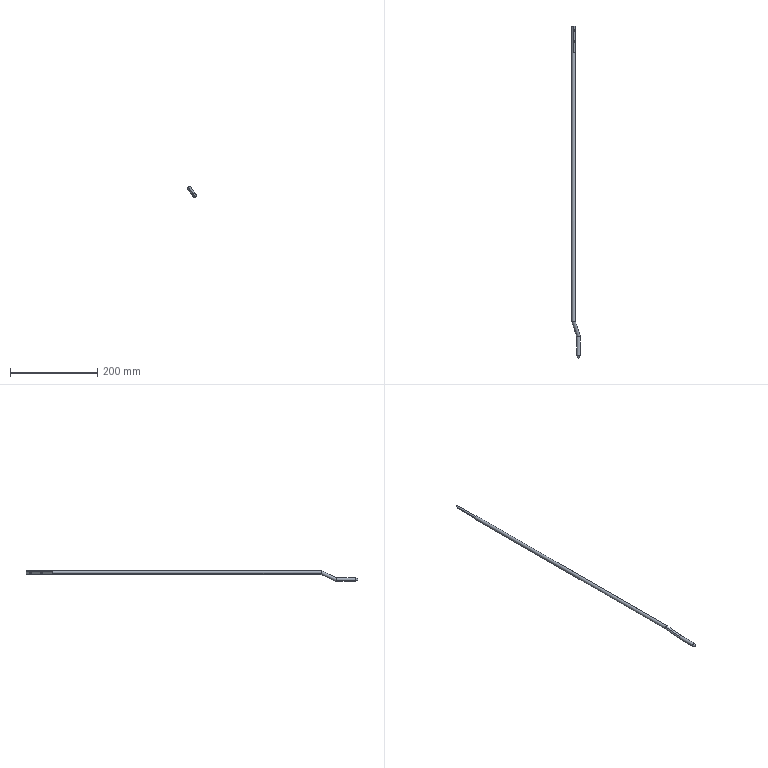Component | SolidWorks | LowerLockRod-1 | 1 solid | 18 faces | box 19.33 x 759.12 x 24.12 mm | volume 36946 mm3 | cylinder 10 | plane 6 | cone 2 | commonest cylinder face diameters 8 x6 4.2 x4
STEP:
#1=CARTESIAN_POINT('',(-12.508,-9.166,84.754));
#2=VERTEX_POINT('',#1);
#3=CARTESIAN_POINT('',(-12.508,-9.332,84.754));
#4=VERTEX_POINT('',#3);
#5=CARTESIAN_POINT('',(-12.508,-9.249,84.754));
#6=DIRECTION('',(-0.818,-0.,-0.5751));
#7=DIRECTION('',(0.,-1.,0.));
#8=AXIS2_PLACEMENT_3D('',#5,#6,#7);
#9=CIRCLE('',#8,0.08268);
#10=EDGE_CURVE('',#2,#4,#9,.T.);
#11=ORIENTED_EDGE('',*,*,#10,.F.);
#12=CARTESIAN_POINT('',(-12.637,-9.166,84.663));
#13=VERTEX_POINT('',#12);
#14=CARTESIAN_POINT('',(-10.705,-9.166,86.022));
#15=DIRECTION('',(-0.818,-0.,-0.5751));
#16=VECTOR('',#15,39.37);
#17=LINE('',#14,#16);
#18=EDGE_CURVE('',#2,#13,#17,.T.);
#19=ORIENTED_EDGE('',*,*,#18,.T.);
#20=CARTESIAN_POINT('',(-12.637,-9.332,84.663));
#21=VERTEX_POINT('',#20);
#22=CARTESIAN_POINT('',(-12.637,-9.249,84.663));
#23=DIRECTION('',(-0.818,-0.,-0.5751));
#24=DIRECTION('',(0.,-1.,0.));
#25=AXIS2_PLACEMENT_3D('',#22,#23,#24);
#26=CIRCLE('',#25,0.08268);
#27=EDGE_CURVE('',#13,#21,#26,.T.);
#28=ORIENTED_EDGE('',*,*,#27,.T.);
#29=CARTESIAN_POINT('',(-10.705,-9.332,86.022));
#30=DIRECTION('',(-0.818,-0.,-0.5751));
#31=VECTOR('',#30,39.37);
#32=LINE('',#29,#31);
#33=EDGE_CURVE('',#4,#21,#32,.T.);
#34=ORIENTED_EDGE('',*,*,#33,.F.);
#35=EDGE_LOOP('',(#11,#19,#28,#34));
#36=FACE_OUTER_BOUND('',#35,.T.);
#37=CARTESIAN_POINT('',(-10.705,-9.249,86.022));
#38=DIRECTION('',(-0.818,-0.,-0.5751));
#39=DIRECTION('',(0.,-1.,0.));
#40=AXIS2_PLACEMENT_3D('',#37,#38,#39);
#41=CYLINDRICAL_SURFACE('',#40,0.08268);
#42=ADVANCED_FACE('',(#36),#41,.F.);
#43=CARTESIAN_POINT('',(-12.508,-8.182,84.754));
#44=VERTEX_POINT('',#43);
#45=CARTESIAN_POINT('',(-12.508,-8.348,84.754));
#46=VERTEX_POINT('',#45);
#47=CARTESIAN_POINT('',(-12.508,-8.265,84.754));
#48=DIRECTION('',(-0.818,-0.,-0.5751));
#49=DIRECTION('',(0.,-1.,0.));
#50=AXIS2_PLACEMENT_3D('',#47,#48,#49);
#51=CIRCLE('',#50,0.08268);
#52=EDGE_CURVE('',#44,#46,#51,.T.);
#53=ORIENTED_EDGE('',*,*,#52,.F.);
#54=CARTESIAN_POINT('',(-12.637,-8.182,84.663));
#55=VERTEX_POINT('',#54);
#56=CARTESIAN_POINT('',(-10.705,-8.182,86.022));
#57=DIRECTION('',(-0.818,-0.,-0.5751));
#58=VECTOR('',#57,39.37);
#59=LINE('',#56,#58);
#60=EDGE_CURVE('',#44,#55,#59,.T.);
#61=ORIENTED_EDGE('',*,*,#60,.T.);
#62=CARTESIAN_POINT('',(-12.637,-8.348,84.663));
#63=VERTEX_POINT('',#62);
#64=CARTESIAN_POINT('',(-12.637,-8.265,84.663));
#65=DIRECTION('',(-0.818,-0.,-0.5751));
#66=DIRECTION('',(0.,-1.,0.));
#67=AXIS2_PLACEMENT_3D('',#64,#65,#66);
#68=CIRCLE('',#67,0.08268);
#69=EDGE_CURVE('',#55,#63,#68,.T.);
#70=ORIENTED_EDGE('',*,*,#69,.T.);
#71=CARTESIAN_POINT('',(-10.705,-8.348,86.022));
#72=DIRECTION('',(-0.818,-0.,-0.5751));
#73=VECTOR('',#72,39.37);
#74=LINE('',#71,#73);
#75=EDGE_CURVE('',#46,#63,#74,.T.);
#76=ORIENTED_EDGE('',*,*,#75,.F.);
#77=EDGE_LOOP('',(#53,#61,#70,#76));
#78=FACE_OUTER_BOUND('',#77,.T.);
#79=CARTESIAN_POINT('',(-10.705,-8.265,86.022));
#80=DIRECTION('',(-0.818,-0.,-0.5751));
#81=DIRECTION('',(0.,-1.,0.));
#82=AXIS2_PLACEMENT_3D('',#79,#80,#81);
#83=CYLINDRICAL_SURFACE('',#82,0.08268);
#84=ADVANCED_FACE('',(#78),#83,.F.);
#85=CARTESIAN_POINT('',(-12.11,-37.758,84.085));
#86=VERTEX_POINT('',#85);
#87=CARTESIAN_POINT('',(-12.143,-37.758,84.063));
#88=VERTEX_POINT('',#87);
#89=CARTESIAN_POINT('',(-12.127,-37.758,84.074));
#90=DIRECTION('',(0.,-1.,-0.));
#91=DIRECTION('',(0.818,0.,0.5751));
#92=AXIS2_PLACEMENT_3D('',#89,#90,#91);
#93=CIRCLE('',#92,0.01969);
#94=EDGE_CURVE('',#86,#88,#93,.T.);
#95=ORIENTED_EDGE('',*,*,#94,.F.);
#96=CARTESIAN_POINT('',(-11.998,-37.522,84.164));
#97=VERTEX_POINT('',#96);
#98=CARTESIAN_POINT('',(-12.11,-37.758,84.085));
#99=DIRECTION('',(0.4122,0.8638,0.2898));
#100=VECTOR('',#99,39.37);
#101=LINE('',#98,#100);
#102=EDGE_CURVE('',#86,#97,#101,.T.);
#103=ORIENTED_EDGE('',*,*,#102,.T.);
#104=CARTESIAN_POINT('',(-12.255,-37.522,83.983));
#105=VERTEX_POINT('',#104);
#106=CARTESIAN_POINT('',(-12.127,-37.522,84.074));
#107=DIRECTION('',(-0.,1.,0.));
#108=DIRECTION('',(0.818,0.,0.5751));
#109=AXIS2_PLACEMENT_3D('',#106,#107,#108);
#110=CIRCLE('',#109,0.1575);
#111=EDGE_CURVE('',#105,#97,#110,.T.);
#112=ORIENTED_EDGE('',*,*,#111,.F.);
#113=CARTESIAN_POINT('',(-12.143,-37.758,84.063));
#114=DIRECTION('',(-0.4122,0.8638,-0.2898));
#115=VECTOR('',#114,39.37);
#116=LINE('',#113,#115);
#117=EDGE_CURVE('',#88,#105,#116,.T.);
#118=ORIENTED_EDGE('',*,*,#117,.F.);
#119=EDGE_LOOP('',(#95,#103,#112,#118));
#120=FACE_OUTER_BOUND('',#119,.T.);
#121=CARTESIAN_POINT('',(-12.127,-37.758,84.074));
#122=DIRECTION('',(-0.,1.,0.));
#123=DIRECTION('',(-0.818,0.,-0.5751));
#124=AXIS2_PLACEMENT_3D('',#121,#122,#123);
#125=CONICAL_SURFACE('',#124,0.01969,0.5281);
#126=ADVANCED_FACE('',(#120),#125,.T.);
#127=CARTESIAN_POINT('',(-12.444,-34.446,84.799));
#128=VERTEX_POINT('',#127);
#129=CARTESIAN_POINT('',(-12.663,-34.488,84.837));
#130=VERTEX_POINT('',#129);
#131=CARTESIAN_POINT('',(-12.444,-34.446,84.799));
#132=CARTESIAN_POINT('',(-12.497,-34.471,84.874));
#133=CARTESIAN_POINT('',(-12.588,-34.488,84.89));
#134=CARTESIAN_POINT('',(-12.663,-34.488,84.837));
#135=(BOUNDED_CURVE()B_SPLINE_CURVE(3,(#131,#132,#133,#134),.UNSPECIFIED.,.F.,.T.)B_SPLINE_CURVE_WITH_KNOTS((4,4),(1.571,3.142),.UNSPECIFIED.)CURVE()GEOMETRIC_REPRESENTATION_ITEM()RATIONAL_B_SPLINE_CURVE((1.,0.8047,0.8047,1.))REPRESENTATION_ITEM(''));
#136=EDGE_CURVE('',#128,#130,#135,.T.);
#137=ORIENTED_EDGE('',*,*,#136,.F.);
#138=CARTESIAN_POINT('',(-12.444,-10.233,84.799));
#139=VERTEX_POINT('',#138);
#140=CARTESIAN_POINT('',(-12.444,-34.891,84.799));
#141=DIRECTION('',(-0.,1.,0.));
#142=VECTOR('',#141,39.37);
#143=LINE('',#140,#142);
#144=EDGE_CURVE('',#128,#139,#143,.T.);
#145=ORIENTED_EDGE('',*,*,#144,.T.);
#146=CARTESIAN_POINT('',(-12.587,-10.233,84.865));
#147=VERTEX_POINT('',#146);
#148=CARTESIAN_POINT('',(-12.573,-10.233,84.708));
#149=DIRECTION('',(-0.,1.,0.));
#150=DIRECTION('',(-0.818,0.,-0.5751));
#151=AXIS2_PLACEMENT_3D('',#148,#149,#150);
#152=CIRCLE('',#151,0.1575);
#153=EDGE_CURVE('',#147,#139,#152,.T.);
#154=ORIENTED_EDGE('',*,*,#153,.F.);
#155=CARTESIAN_POINT('',(-12.587,-7.871,84.865));
#156=VERTEX_POINT('',#155);
#157=CARTESIAN_POINT('',(-12.587,-10.233,84.865));
#158=DIRECTION('',(-0.,1.,0.));
#159=VECTOR('',#158,39.37);
#160=LINE('',#157,#159);
#161=EDGE_CURVE('',#147,#156,#160,.T.);
#162=ORIENTED_EDGE('',*,*,#161,.T.);
#163=CARTESIAN_POINT('',(-12.716,-7.871,84.775));
#164=VERTEX_POINT('',#163);
#165=CARTESIAN_POINT('',(-12.573,-7.871,84.708));
#166=DIRECTION('',(0.,-1.,-0.));
#167=DIRECTION('',(0.818,0.,0.5751));
#168=AXIS2_PLACEMENT_3D('',#165,#166,#167);
#169=CIRCLE('',#168,0.1575);
#170=EDGE_CURVE('',#156,#164,#169,.T.);
#171=ORIENTED_EDGE('',*,*,#170,.T.);
#172=CARTESIAN_POINT('',(-12.716,-10.233,84.775));
#173=VERTEX_POINT('',#172);
#174=CARTESIAN_POINT('',(-12.716,-10.233,84.775));
#175=DIRECTION('',(-0.,1.,0.));
#176=VECTOR('',#175,39.37);
#177=LINE('',#174,#176);
#178=EDGE_CURVE('',#173,#164,#177,.T.);
#179=ORIENTED_EDGE('',*,*,#178,.F.);
#180=CARTESIAN_POINT('',(-12.701,-10.233,84.618));
#181=VERTEX_POINT('',#180);
#182=CARTESIAN_POINT('',(-12.573,-10.233,84.708));
#183=DIRECTION('',(-0.,1.,0.));
#184=DIRECTION('',(-0.818,0.,-0.5751));
#185=AXIS2_PLACEMENT_3D('',#182,#183,#184);
#186=CIRCLE('',#185,0.1575);
#187=EDGE_CURVE('',#181,#173,#186,.T.);
#188=ORIENTED_EDGE('',*,*,#187,.F.);
#189=CARTESIAN_POINT('',(-12.701,-34.446,84.618));
#190=VERTEX_POINT('',#189);
#191=CARTESIAN_POINT('',(-12.701,-34.891,84.618));
#192=DIRECTION('',(-0.,1.,0.));
#193=VECTOR('',#192,39.37);
#194=LINE('',#191,#193);
#195=EDGE_CURVE('',#190,#181,#194,.T.);
#196=ORIENTED_EDGE('',*,*,#195,.F.);
#197=CARTESIAN_POINT('',(-12.663,-34.488,84.837));
#198=CARTESIAN_POINT('',(-12.739,-34.488,84.784));
#199=CARTESIAN_POINT('',(-12.755,-34.471,84.693));
#200=CARTESIAN_POINT('',(-12.701,-34.446,84.618));
#201=(BOUNDED_CURVE()B_SPLINE_CURVE(3,(#197,#198,#199,#200),.UNSPECIFIED.,.F.,.T.)B_SPLINE_CURVE_WITH_KNOTS((4,4),(3.142,4.712),.UNSPECIFIED.)CURVE()GEOMETRIC_REPRESENTATION_ITEM()RATIONAL_B_SPLINE_CURVE((1.,0.8047,0.8047,1.))REPRESENTATION_ITEM(''));
#202=EDGE_CURVE('',#130,#190,#201,.T.);
#203=ORIENTED_EDGE('',*,*,#202,.F.);
#204=EDGE_LOOP('',(#137,#145,#154,#162,#171,#179,#188,#196,#203));
#205=FACE_OUTER_BOUND('',#204,.T.);
#206=CARTESIAN_POINT('',(-12.573,-34.891,84.708));
#207=DIRECTION('',(-0.,1.,0.));
#208=DIRECTION('',(-0.818,0.,-0.5751));
#209=AXIS2_PLACEMENT_3D('',#206,#207,#208);
#210=CYLINDRICAL_SURFACE('',#209,0.1575);
#211=ADVANCED_FACE('',(#205),#210,.T.);
#212=ORIENTED_EDGE('',*,*,#202,.T.);
#213=CARTESIAN_POINT('',(-12.482,-34.404,84.58));
#214=VERTEX_POINT('',#213);
#215=CARTESIAN_POINT('',(-12.701,-34.446,84.618));
#216=CARTESIAN_POINT('',(-12.648,-34.421,84.542));
#217=CARTESIAN_POINT('',(-12.558,-34.404,84.527));
#218=CARTESIAN_POINT('',(-12.482,-34.404,84.58));
#219=(BOUNDED_CURVE()B_SPLINE_CURVE(3,(#215,#216,#217,#218),.UNSPECIFIED.,.F.,.T.)B_SPLINE_CURVE_WITH_KNOTS((4,4),(4.712,6.283),.UNSPECIFIED.)CURVE()GEOMETRIC_REPRESENTATION_ITEM()RATIONAL_B_SPLINE_CURVE((1.,0.8047,0.8047,1.))REPRESENTATION_ITEM(''));
#220=EDGE_CURVE('',#190,#214,#219,.T.);
#221=ORIENTED_EDGE('',*,*,#220,.T.);
#222=CARTESIAN_POINT('',(-12.036,-35.747,83.945));
#223=VERTEX_POINT('',#222);
#224=CARTESIAN_POINT('',(-12.494,-34.367,84.597));
#225=DIRECTION('',(0.2876,-0.866,-0.409));
#226=VECTOR('',#225,39.37);
#227=LINE('',#224,#226);
#228=EDGE_CURVE('',#214,#223,#227,.T.);
#229=ORIENTED_EDGE('',*,*,#228,.T.);
#230=CARTESIAN_POINT('',(-12.255,-35.789,83.983));
#231=VERTEX_POINT('',#230);
#232=CARTESIAN_POINT('',(-12.036,-35.747,83.945));
#233=CARTESIAN_POINT('',(-12.111,-35.747,83.892));
#234=CARTESIAN_POINT('',(-12.202,-35.765,83.908));
#235=CARTESIAN_POINT('',(-12.255,-35.789,83.983));
#236=(BOUNDED_CURVE()B_SPLINE_CURVE(3,(#232,#233,#234,#235),.UNSPECIFIED.,.F.,.F.)B_SPLINE_CURVE_WITH_KNOTS((4,4),(0.,1.571),.UNSPECIFIED.)CURVE()GEOMETRIC_REPRESENTATION_ITEM()RATIONAL_B_SPLINE_CURVE((1.,0.8047,0.8047,1.))REPRESENTATION_ITEM(''));
#237=EDGE_CURVE('',#223,#231,#236,.T.);
#238=ORIENTED_EDGE('',*,*,#237,.T.);
#239=CARTESIAN_POINT('',(-12.217,-35.832,84.203));
#240=VERTEX_POINT('',#239);
#241=CARTESIAN_POINT('',(-12.255,-35.789,83.983));
#242=CARTESIAN_POINT('',(-12.308,-35.814,84.059));
#243=CARTESIAN_POINT('',(-12.293,-35.832,84.15));
#244=CARTESIAN_POINT('',(-12.217,-35.832,84.203));
#245=(BOUNDED_CURVE()B_SPLINE_CURVE(3,(#241,#242,#243,#244),.UNSPECIFIED.,.F.,.T.)B_SPLINE_CURVE_WITH_KNOTS((4,4),(1.571,3.142),.UNSPECIFIED.)CURVE()GEOMETRIC_REPRESENTATION_ITEM()RATIONAL_B_SPLINE_CURVE((1.,0.8047,0.8047,1.))REPRESENTATION_ITEM(''));
#246=EDGE_CURVE('',#231,#240,#245,.T.);
#247=ORIENTED_EDGE('',*,*,#246,.T.);
#248=CARTESIAN_POINT('',(-12.651,-34.525,84.82));
#249=DIRECTION('',(0.2876,-0.866,-0.409));
#250=VECTOR('',#249,39.37);
#251=LINE('',#248,#250);
#252=EDGE_CURVE('',#130,#240,#251,.T.);
#253=ORIENTED_EDGE('',*,*,#252,.F.);
#254=EDGE_LOOP('',(#212,#221,#229,#238,#247,#253));
#255=FACE_OUTER_BOUND('',#254,.T.);
#256=CARTESIAN_POINT('',(-12.573,-34.446,84.708));
#257=DIRECTION('',(0.2876,-0.866,-0.409));
#258=DIRECTION('',(-0.4981,-0.5,0.7085));
#259=AXIS2_PLACEMENT_3D('',#256,#257,#258);
#260=CYLINDRICAL_SURFACE('',#259,0.1575);
#261=ADVANCED_FACE('',(#255),#260,.T.);
#262=ORIENTED_EDGE('',*,*,#246,.F.);
#263=CARTESIAN_POINT('',(-12.255,-35.789,83.983));
#264=DIRECTION('',(0.,-1.,-0.));
#265=VECTOR('',#264,39.37);
#266=LINE('',#263,#265);
#267=EDGE_CURVE('',#231,#105,#266,.T.);
#268=ORIENTED_EDGE('',*,*,#267,.T.);
#269=ORIENTED_EDGE('',*,*,#111,.T.);
#270=CARTESIAN_POINT('',(-11.998,-35.789,84.164));
#271=VERTEX_POINT('',#270);
#272=CARTESIAN_POINT('',(-11.998,-35.789,84.164));
#273=DIRECTION('',(0.,-1.,-0.));
#274=VECTOR('',#273,39.37);
#275=LINE('',#272,#274);
#276=EDGE_CURVE('',#271,#97,#275,.T.);
#277=ORIENTED_EDGE('',*,*,#276,.F.);
#278=CARTESIAN_POINT('',(-12.217,-35.832,84.203));
#279=CARTESIAN_POINT('',(-12.142,-35.832,84.256));
#280=CARTESIAN_POINT('',(-12.051,-35.814,84.24));
#281=CARTESIAN_POINT('',(-11.998,-35.789,84.164));
#282=(BOUNDED_CURVE()B_SPLINE_CURVE(3,(#278,#279,#280,#281),.UNSPECIFIED.,.F.,.T.)B_SPLINE_CURVE_WITH_KNOTS((4,4),(3.142,4.712),.UNSPECIFIED.)CURVE()GEOMETRIC_REPRESENTATION_ITEM()RATIONAL_B_SPLINE_CURVE((1.,0.8047,0.8047,1.))REPRESENTATION_ITEM(''));
#283=EDGE_CURVE('',#240,#271,#282,.T.);
#284=ORIENTED_EDGE('',*,*,#283,.F.);
#285=EDGE_LOOP('',(#262,#268,#269,#277,#284));
#286=FACE_OUTER_BOUND('',#285,.T.);
#287=CARTESIAN_POINT('',(-12.127,-35.789,84.074));
#288=DIRECTION('',(0.,-1.,-0.));
#289=DIRECTION('',(0.818,0.,0.5751));
#290=AXIS2_PLACEMENT_3D('',#287,#288,#289);
#291=CYLINDRICAL_SURFACE('',#290,0.1575);
#292=ADVANCED_FACE('',(#286),#291,.T.);
#293=ORIENTED_EDGE('',*,*,#267,.F.);
#294=ORIENTED_EDGE('',*,*,#237,.F.);
#295=CARTESIAN_POINT('',(-11.998,-35.789,84.164));
#296=CARTESIAN_POINT('',(-11.945,-35.765,84.089));
#297=CARTESIAN_POINT('',(-11.961,-35.747,83.998));
#298=CARTESIAN_POINT('',(-12.036,-35.747,83.945));
#299=(BOUNDED_CURVE()B_SPLINE_CURVE(3,(#295,#296,#297,#298),.UNSPECIFIED.,.F.,.T.)B_SPLINE_CURVE_WITH_KNOTS((4,4),(4.712,6.283),.UNSPECIFIED.)CURVE()GEOMETRIC_REPRESENTATION_ITEM()RATIONAL_B_SPLINE_CURVE((1.,0.8047,0.8047,1.))REPRESENTATION_ITEM(''));
#300=EDGE_CURVE('',#271,#223,#299,.T.);
#301=ORIENTED_EDGE('',*,*,#300,.F.);
#302=ORIENTED_EDGE('',*,*,#276,.T.);
#303=CARTESIAN_POINT('',(-12.127,-37.522,84.074));
#304=DIRECTION('',(-0.,1.,0.));
#305=DIRECTION('',(0.818,0.,0.5751));
#306=AXIS2_PLACEMENT_3D('',#303,#304,#305);
#307=CIRCLE('',#306,0.1575);
#308=EDGE_CURVE('',#97,#105,#307,.T.);
#309=ORIENTED_EDGE('',*,*,#308,.T.);
#310=EDGE_LOOP('',(#293,#294,#301,#302,#309));
#311=FACE_OUTER_BOUND('',#310,.T.);
#312=CARTESIAN_POINT('',(-12.127,-35.789,84.074));
#313=DIRECTION('',(0.,-1.,-0.));
#314=DIRECTION('',(0.818,0.,0.5751));
#315=AXIS2_PLACEMENT_3D('',#312,#313,#314);
#316=CYLINDRICAL_SURFACE('',#315,0.1575);
#317=ADVANCED_FACE('',(#311),#316,.T.);
#318=ORIENTED_EDGE('',*,*,#228,.F.);
#319=CARTESIAN_POINT('',(-12.482,-34.404,84.58));
#320=CARTESIAN_POINT('',(-12.407,-34.404,84.633));
#321=CARTESIAN_POINT('',(-12.391,-34.421,84.724));
#322=CARTESIAN_POINT('',(-12.444,-34.446,84.799));
#323=(BOUNDED_CURVE()B_SPLINE_CURVE(3,(#319,#320,#321,#322),.UNSPECIFIED.,.F.,.T.)B_SPLINE_CURVE_WITH_KNOTS((4,4),(-0.,1.571),.UNSPECIFIED.)CURVE()GEOMETRIC_REPRESENTATION_ITEM()RATIONAL_B_SPLINE_CURVE((1.,0.8047,0.8047,1.))REPRESENTATION_ITEM(''));
#324=EDGE_CURVE('',#214,#128,#323,.T.);
#325=ORIENTED_EDGE('',*,*,#324,.T.);
#326=ORIENTED_EDGE('',*,*,#136,.T.);
#327=ORIENTED_EDGE('',*,*,#252,.T.);
#328=ORIENTED_EDGE('',*,*,#283,.T.);
#329=ORIENTED_EDGE('',*,*,#300,.T.);
#330=EDGE_LOOP('',(#318,#325,#326,#327,#328,#329));
#331=FACE_OUTER_BOUND('',#330,.T.);
#332=CARTESIAN_POINT('',(-12.573,-34.446,84.708));
#333=DIRECTION('',(0.2876,-0.866,-0.409));
#334=DIRECTION('',(-0.4981,-0.5,0.7085));
#335=AXIS2_PLACEMENT_3D('',#332,#333,#334);
#336=CYLINDRICAL_SURFACE('',#335,0.1575);
#337=ADVANCED_FACE('',(#331),#336,.T.);
#338=ORIENTED_EDGE('',*,*,#144,.F.);
#339=ORIENTED_EDGE('',*,*,#324,.F.);
#340=ORIENTED_EDGE('',*,*,#220,.F.);
#341=ORIENTED_EDGE('',*,*,#195,.T.);
#342=CARTESIAN_POINT('',(-12.559,-10.233,84.552));
#343=VERTEX_POINT('',#342);
#344=CARTESIAN_POINT('',(-12.573,-10.233,84.708));
#345=DIRECTION('',(-0.,1.,0.));
#346=DIRECTION('',(-0.818,0.,-0.5751));
#347=AXIS2_PLACEMENT_3D('',#344,#345,#346);
#348=CIRCLE('',#347,0.1575);
#349=EDGE_CURVE('',#343,#181,#348,.T.);
#350=ORIENTED_EDGE('',*,*,#349,.F.);
#351=CARTESIAN_POINT('',(-12.559,-7.871,84.552));
#352=VERTEX_POINT('',#351);
#353=CARTESIAN_POINT('',(-12.559,-10.233,84.552));
#354=DIRECTION('',(-0.,1.,0.));
#355=VECTOR('',#354,39.37);
#356=LINE('',#353,#355);
#357=EDGE_CURVE('',#343,#352,#356,.T.);
#358=ORIENTED_EDGE('',*,*,#357,.T.);
#359=CARTESIAN_POINT('',(-12.43,-7.871,84.642));
#360=VERTEX_POINT('',#359);
#361=CARTESIAN_POINT('',(-12.573,-7.871,84.708));
#362=DIRECTION('',(0.,-1.,-0.));
#363=DIRECTION('',(0.818,0.,0.5751));
#364=AXIS2_PLACEMENT_3D('',#361,#362,#363);
#365=CIRCLE('',#364,0.1575);
#366=EDGE_CURVE('',#352,#360,#365,.T.);
#367=ORIENTED_EDGE('',*,*,#366,.T.);
#368=CARTESIAN_POINT('',(-12.43,-10.233,84.642));
#369=VERTEX_POINT('',#368);
#370=CARTESIAN_POINT('',(-12.43,-10.233,84.642));
#371=DIRECTION('',(-0.,1.,0.));
#372=VECTOR('',#371,39.37);
#373=LINE('',#370,#372);
#374=EDGE_CURVE('',#369,#360,#373,.T.);
#375=ORIENTED_EDGE('',*,*,#374,.F.);
#376=CARTESIAN_POINT('',(-12.573,-10.233,84.708));
#377=DIRECTION('',(-0.,1.,0.));
#378=DIRECTION('',(-0.818,0.,-0.5751));
#379=AXIS2_PLACEMENT_3D('',#376,#377,#378);
#380=CIRCLE('',#379,0.1575);
#381=EDGE_CURVE('',#139,#369,#380,.T.);
#382=ORIENTED_EDGE('',*,*,#381,.F.);
#383=EDGE_LOOP('',(#338,#339,#340,#341,#350,#358,#367,#375,#382));
#384=FACE_OUTER_BOUND('',#383,.T.);
#385=CARTESIAN_POINT('',(-12.573,-34.891,84.708));
#386=DIRECTION('',(-0.,1.,0.));
#387=DIRECTION('',(-0.818,0.,-0.5751));
#388=AXIS2_PLACEMENT_3D('',#385,#386,#387);
#389=CYLINDRICAL_SURFACE('',#388,0.1575);
#390=ADVANCED_FACE('',(#384),#389,.T.);
#391=ORIENTED_EDGE('',*,*,#170,.F.);
#392=CARTESIAN_POINT('',(-12.587,-7.871,84.865));
#393=DIRECTION('',(-0.5751,-0.,0.818));
#394=VECTOR('',#393,39.37);
#395=LINE('',#392,#394);
#396=EDGE_CURVE('',#360,#156,#395,.T.);
#397=ORIENTED_EDGE('',*,*,#396,.F.);
#398=ORIENTED_EDGE('',*,*,#366,.F.);
#399=CARTESIAN_POINT('',(-12.716,-7.871,84.775));
#400=DIRECTION('',(0.5751,0.,-0.818));
#401=VECTOR('',#400,39.37);
#402=LINE('',#399,#401);
#403=EDGE_CURVE('',#164,#352,#402,.T.);
#404=ORIENTED_EDGE('',*,*,#403,.F.);
#405=EDGE_LOOP('',(#391,#397,#398,#404));
#406=FACE_OUTER_BOUND('',#405,.T.);
#407=CARTESIAN_POINT('',(-12.573,-7.871,84.708));
#408=DIRECTION('',(0.,-1.,-0.));
#409=DIRECTION('',(0.818,0.,0.5751));
#410=AXIS2_PLACEMENT_3D('',#407,#408,#409);
#411=PLANE('',#410);
#412=ADVANCED_FACE('',(#406),#411,.F.);
#413=CARTESIAN_POINT('',(-12.127,-37.758,84.074));
#414=DIRECTION('',(0.,-1.,-0.));
#415=DIRECTION('',(0.818,0.,0.5751));
#416=AXIS2_PLACEMENT_3D('',#413,#414,#415);
#417=CIRCLE('',#416,0.01969);
#418=EDGE_CURVE('',#88,#86,#417,.T.);
#419=ORIENTED_EDGE('',*,*,#418,.T.);
#420=ORIENTED_EDGE('',*,*,#94,.T.);
#421=EDGE_LOOP('',(#419,#420));
#422=FACE_OUTER_BOUND('',#421,.T.);
#423=CARTESIAN_POINT('',(-12.127,-37.758,84.074));
#424=DIRECTION('',(0.,-1.,-0.));
#425=DIRECTION('',(0.818,0.,0.5751));
#426=AXIS2_PLACEMENT_3D('',#423,#424,#425);
#427=PLANE('',#426);
#428=ADVANCED_FACE('',(#422),#427,.T.);
#429=ORIENTED_EDGE('',*,*,#102,.F.);
#430=ORIENTED_EDGE('',*,*,#418,.F.);
#431=ORIENTED_EDGE('',*,*,#117,.T.);
#432=ORIENTED_EDGE('',*,*,#308,.F.);
#433=EDGE_LOOP('',(#429,#430,#431,#432));
#434=FACE_OUTER_BOUND('',#433,.T.);
#435=CARTESIAN_POINT('',(-12.127,-37.758,84.074));
#436=DIRECTION('',(-0.,1.,0.));
#437=DIRECTION('',(-0.818,0.,-0.5751));
#438=AXIS2_PLACEMENT_3D('',#435,#436,#437);
#439=CONICAL_SURFACE('',#438,0.01969,0.5281);
#440=ADVANCED_FACE('',(#434),#439,.T.);
#441=CARTESIAN_POINT('',(-12.637,-9.249,84.663));
#442=DIRECTION('',(-0.818,-0.,-0.5751));
#443=DIRECTION('',(0.,-1.,0.));
#444=AXIS2_PLACEMENT_3D('',#441,#442,#443);
#445=CIRCLE('',#444,0.08268);
#446=EDGE_CURVE('',#21,#13,#445,.T.);
#447=ORIENTED_EDGE('',*,*,#446,.F.);
#448=ORIENTED_EDGE('',*,*,#27,.F.);
#449=EDGE_LOOP('',(#447,#448));
#450=FACE_BOUND('',#449,.T.);
#451=CARTESIAN_POINT('',(-12.637,-8.265,84.663));
#452=DIRECTION('',(-0.818,-0.,-0.5751));
#453=DIRECTION('',(0.,-1.,0.));
#454=AXIS2_PLACEMENT_3D('',#451,#452,#453);
#455=CIRCLE('',#454,0.08268);
#456=EDGE_CURVE('',#63,#55,#455,.T.);
#457=ORIENTED_EDGE('',*,*,#456,.F.);
#458=ORIENTED_EDGE('',*,*,#69,.F.);
#459=EDGE_LOOP('',(#457,#458));
#460=FACE_BOUND('',#459,.T.);
#461=ORIENTED_EDGE('',*,*,#403,.T.);
#462=ORIENTED_EDGE('',*,*,#357,.F.);
#463=CARTESIAN_POINT('',(-12.716,-10.233,84.775));
#464=DIRECTION('',(0.5751,0.,-0.818));
#465=VECTOR('',#464,39.37);
#466=LINE('',#463,#465);
#467=EDGE_CURVE('',#173,#343,#466,.T.);
#468=ORIENTED_EDGE('',*,*,#467,.F.);
#469=ORIENTED_EDGE('',*,*,#178,.T.);
#470=EDGE_LOOP('',(#461,#462,#468,#469));
#471=FACE_OUTER_BOUND('',#470,.T.);
#472=CARTESIAN_POINT('',(-12.716,-10.233,84.775));
#473=DIRECTION('',(0.818,0.,0.5751));
#474=DIRECTION('',(-0.,1.,0.));
#475=AXIS2_PLACEMENT_3D('',#472,#473,#474);
#476=PLANE('',#475);
#477=ADVANCED_FACE('',(#450,#460,#471),#476,.F.);
#478=ORIENTED_EDGE('',*,*,#349,.T.);
#479=ORIENTED_EDGE('',*,*,#187,.T.);
#480=ORIENTED_EDGE('',*,*,#467,.T.);
#481=EDGE_LOOP('',(#478,#479,#480));
#482=FACE_OUTER_BOUND('',#481,.T.);
#483=CARTESIAN_POINT('',(-12.573,-10.233,84.708));
#484=DIRECTION('',(-0.,1.,0.));
#485=DIRECTION('',(-0.818,-0.,-0.5751));
#486=AXIS2_PLACEMENT_3D('',#483,#484,#485);
#487=PLANE('',#486);
#488=ADVANCED_FACE('',(#482),#487,.T.);
#489=CARTESIAN_POINT('',(-12.508,-9.249,84.754));
#490=DIRECTION('',(-0.818,-0.,-0.5751));
#491=DIRECTION('',(0.,-1.,0.));
#492=AXIS2_PLACEMENT_3D('',#489,#490,#491);
#493=CIRCLE('',#492,0.08268);
#494=EDGE_CURVE('',#4,#2,#493,.T.);
#495=ORIENTED_EDGE('',*,*,#494,.T.);
#496=ORIENTED_EDGE('',*,*,#10,.T.);
#497=EDGE_LOOP('',(#495,#496));
#498=FACE_BOUND('',#497,.T.);
#499=CARTESIAN_POINT('',(-12.508,-8.265,84.754));
#500=DIRECTION('',(-0.818,-0.,-0.5751));
#501=DIRECTION('',(0.,-1.,0.));
#502=AXIS2_PLACEMENT_3D('',#499,#500,#501);
#503=CIRCLE('',#502,0.08268);
#504=EDGE_CURVE('',#46,#44,#503,.T.);
#505=ORIENTED_EDGE('',*,*,#504,.T.);
#506=ORIENTED_EDGE('',*,*,#52,.T.);
#507=EDGE_LOOP('',(#505,#506));
#508=FACE_BOUND('',#507,.T.);
#509=ORIENTED_EDGE('',*,*,#396,.T.);
#510=ORIENTED_EDGE('',*,*,#161,.F.);
#511=CARTESIAN_POINT('',(-12.587,-10.233,84.865));
#512=DIRECTION('',(-0.5751,-0.,0.818));
#513=VECTOR('',#512,39.37);
#514=LINE('',#511,#513);
#515=EDGE_CURVE('',#369,#147,#514,.T.);
#516=ORIENTED_EDGE('',*,*,#515,.F.);
#517=ORIENTED_EDGE('',*,*,#374,.T.);
#518=EDGE_LOOP('',(#509,#510,#516,#517));
#519=FACE_OUTER_BOUND('',#518,.T.);
#520=CARTESIAN_POINT('',(-12.587,-10.233,84.865));
#521=DIRECTION('',(-0.818,-0.,-0.5751));
#522=DIRECTION('',(0.,-1.,-0.));
#523=AXIS2_PLACEMENT_3D('',#520,#521,#522);
#524=PLANE('',#523);
#525=ADVANCED_FACE('',(#498,#508,#519),#524,.F.);
#526=ORIENTED_EDGE('',*,*,#153,.T.);
#527=ORIENTED_EDGE('',*,*,#381,.T.);
#528=ORIENTED_EDGE('',*,*,#515,.T.);
#529=EDGE_LOOP('',(#526,#527,#528));
#530=FACE_OUTER_BOUND('',#529,.T.);
#531=CARTESIAN_POINT('',(-12.573,-10.233,84.708));
#532=DIRECTION('',(-0.,1.,0.));
#533=DIRECTION('',(-0.818,-0.,-0.5751));
#534=AXIS2_PLACEMENT_3D('',#531,#532,#533);
#535=PLANE('',#534);
#536=ADVANCED_FACE('',(#530),#535,.T.);
#537=ORIENTED_EDGE('',*,*,#60,.F.);
#538=ORIENTED_EDGE('',*,*,#504,.F.);
#539=ORIENTED_EDGE('',*,*,#75,.T.);
#540=ORIENTED_EDGE('',*,*,#456,.T.);
#541=EDGE_LOOP('',(#537,#538,#539,#540));
#542=FACE_OUTER_BOUND('',#541,.T.);
#543=CARTESIAN_POINT('',(-10.705,-8.265,86.022));
#544=DIRECTION('',(-0.818,-0.,-0.5751));
#545=DIRECTION('',(0.,-1.,0.));
#546=AXIS2_PLACEMENT_3D('',#543,#544,#545);
#547=CYLINDRICAL_SURFACE('',#546,0.08268);
#548=ADVANCED_FACE('',(#542),#547,.F.);
#549=ORIENTED_EDGE('',*,*,#18,.F.);
#550=ORIENTED_EDGE('',*,*,#494,.F.);
#551=ORIENTED_EDGE('',*,*,#33,.T.);
#552=ORIENTED_EDGE('',*,*,#446,.T.);
#553=EDGE_LOOP('',(#549,#550,#551,#552));
#554=FACE_OUTER_BOUND('',#553,.T.);
#555=CARTESIAN_POINT('',(-10.705,-9.249,86.022));
#556=DIRECTION('',(-0.818,-0.,-0.5751));
#557=DIRECTION('',(0.,-1.,0.));
#558=AXIS2_PLACEMENT_3D('',#555,#556,#557);
#559=CYLINDRICAL_SURFACE('',#558,0.08268);
#560=ADVANCED_FACE('',(#554),#559,.F.);
#561=CLOSED_SHELL('',(#42,#84,#126,#211,#261,#292,#317,#337,#390,#412,#428,#440,#477,#488,#525,#536,#548,#560));
#562=MANIFOLD_SOLID_BREP('',#561);
#563=CARTESIAN_POINT('',(0.,0.,0.));
#564=DIRECTION('',(0.,0.,1.));
#565=DIRECTION('',(1.,0.,0.));
#566=AXIS2_PLACEMENT_3D('',#563,#564,#565);
#567=(LENGTH_UNIT()NAMED_UNIT(*)SI_UNIT($,.METRE.));
#568=LENGTH_MEASURE_WITH_UNIT(LENGTH_MEASURE(0.0254),#567);
#569=DIMENSIONAL_EXPONENTS(1.,0.,0.,0.,0.,0.,0.);
#570=(CONVERSION_BASED_UNIT('',#568)LENGTH_UNIT()NAMED_UNIT(#569));
#571=UNCERTAINTY_MEASURE_WITH_UNIT(LENGTH_MEASURE(0.00001),#570,'','');
#572=(NAMED_UNIT(*)PLANE_ANGLE_UNIT()SI_UNIT($,.RADIAN.));
#573=(NAMED_UNIT(*)SI_UNIT($,.STERADIAN.)SOLID_ANGLE_UNIT());
#574=(GEOMETRIC_REPRESENTATION_CONTEXT(3)GLOBAL_UNCERTAINTY_ASSIGNED_CONTEXT((#571))GLOBAL_UNIT_ASSIGNED_CONTEXT((#570,#572,#573))REPRESENTATION_CONTEXT('',''));
#575=ADVANCED_BREP_SHAPE_REPRESENTATION('',(#562,#566),#574);
#576=COLOUR_RGB('',0.7922,0.8196,0.9333);
#577=FILL_AREA_STYLE_COLOUR('',#576);
#578=FILL_AREA_STYLE('',(#577));
#579=SURFACE_STYLE_FILL_AREA(#578);
#580=SURFACE_SIDE_STYLE('',(#579));
#581=SURFACE_STYLE_USAGE(.BOTH.,#580);
#582=PRESENTATION_STYLE_ASSIGNMENT((#581));
#583=STYLED_ITEM('',(#582),#562);
#584=(LENGTH_UNIT()NAMED_UNIT(*)SI_UNIT($,.METRE.));
#585=LENGTH_MEASURE_WITH_UNIT(LENGTH_MEASURE(0.0254),#584);
#586=DIMENSIONAL_EXPONENTS(1.,0.,0.,0.,0.,0.,0.);
#587=(CONVERSION_BASED_UNIT('',#585)LENGTH_UNIT()NAMED_UNIT(#586));
#588=UNCERTAINTY_MEASURE_WITH_UNIT(LENGTH_MEASURE(0.00001),#587,'','');
#589=(NAMED_UNIT(*)PLANE_ANGLE_UNIT()SI_UNIT($,.RADIAN.));
#590=(NAMED_UNIT(*)SI_UNIT($,.STERADIAN.)SOLID_ANGLE_UNIT());
#591=(GEOMETRIC_REPRESENTATION_CONTEXT(3)GLOBAL_UNCERTAINTY_ASSIGNED_CONTEXT((#588))GLOBAL_UNIT_ASSIGNED_CONTEXT((#587,#589,#590))REPRESENTATION_CONTEXT('',''));
#592=MECHANICAL_DESIGN_GEOMETRIC_PRESENTATION_REPRESENTATION('',(#583),#591);
#593=PRESENTATION_LAYER_ASSIGNMENT('','',(#583));